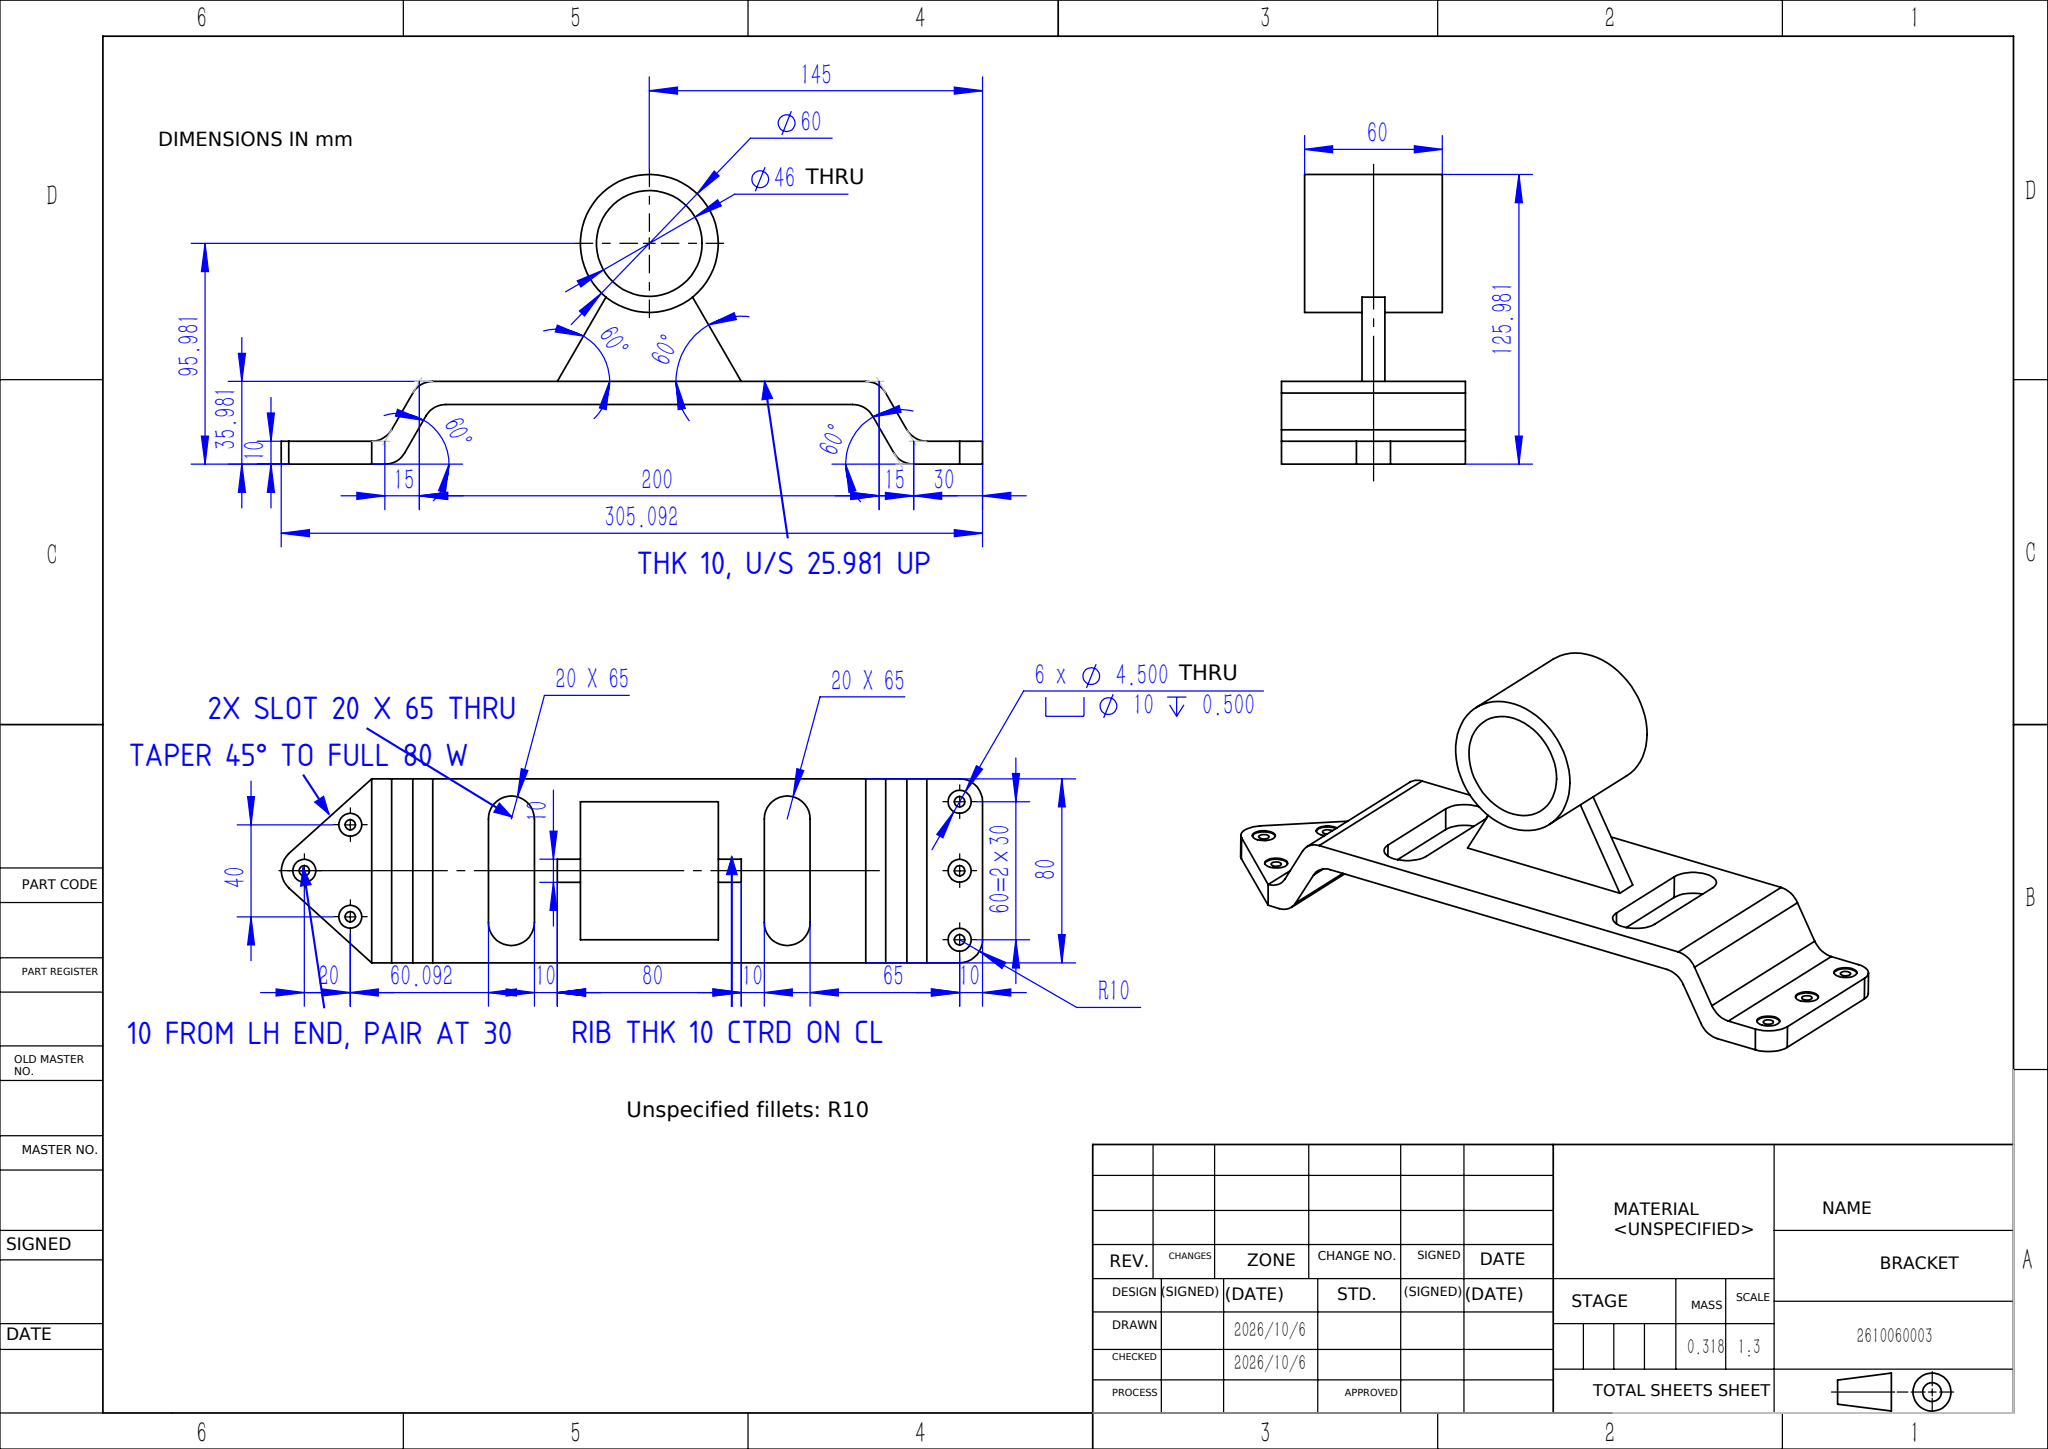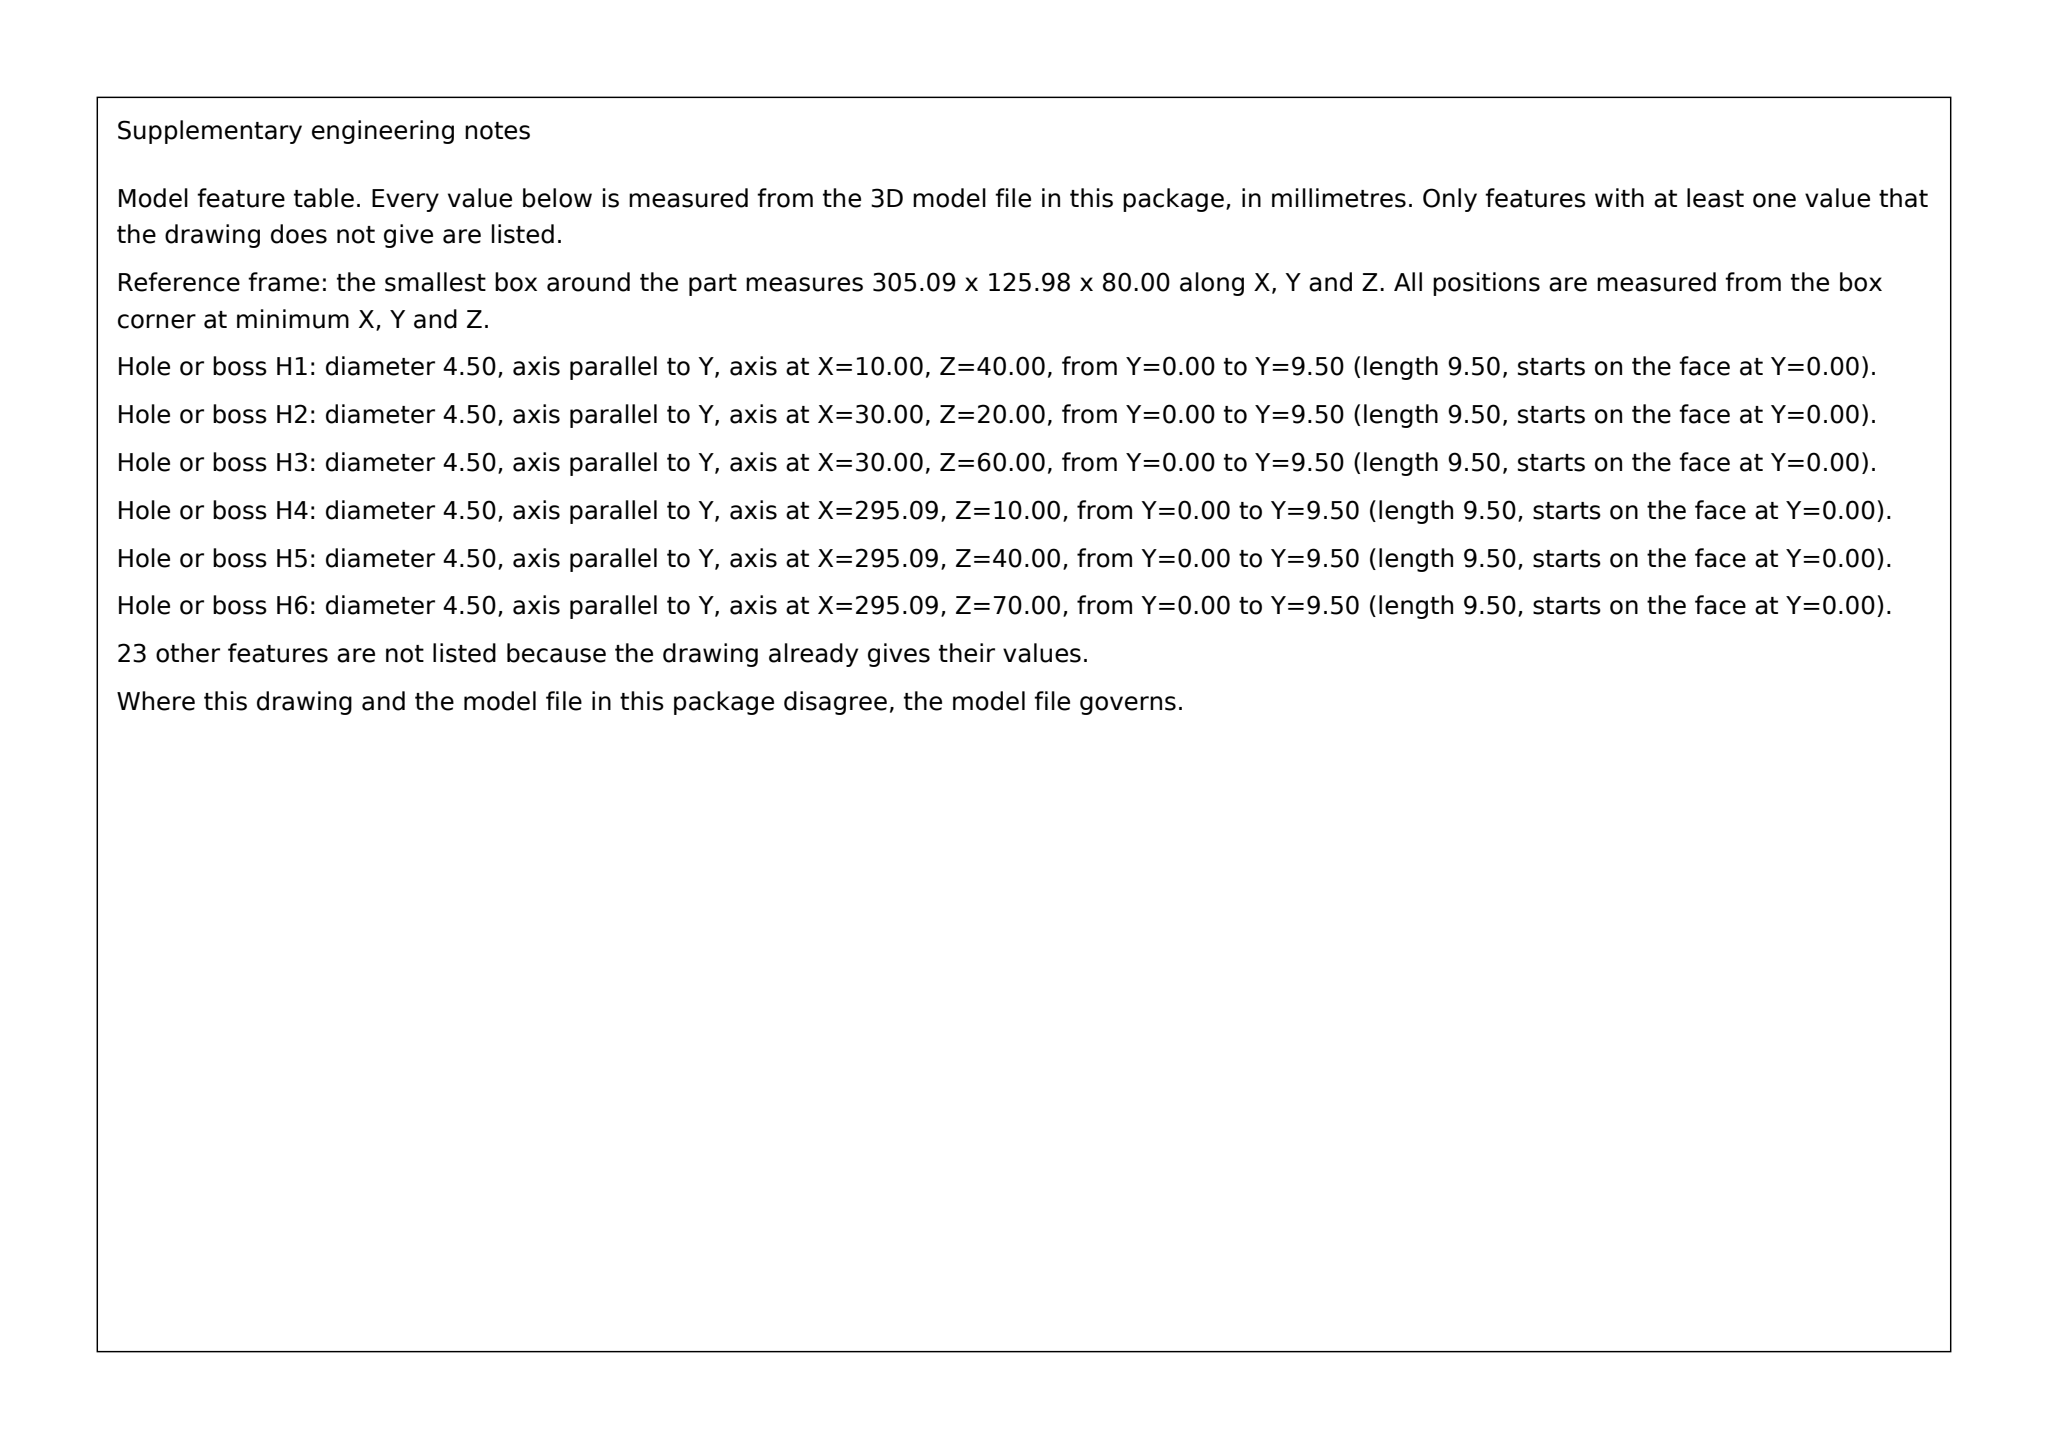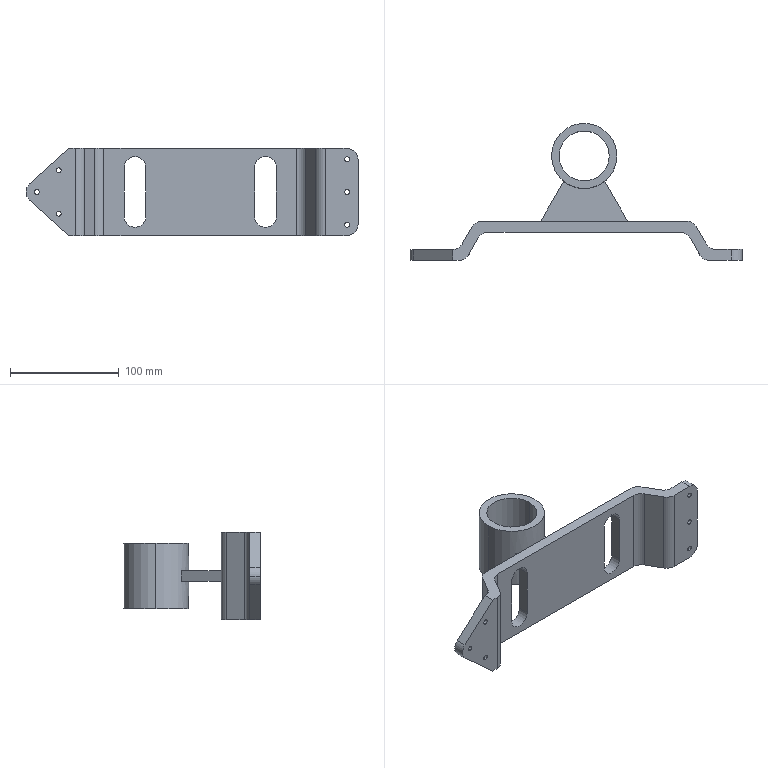Part | SolidWorks | mm | 1 solid | 77 faces | box 305.09 x 125.98 x 80 mm | volume 317970 mm3 | cylinder 46 | plane 31 | commonest cylinder face diameters 20 x18 10 x12 4.5 x12 46 x2 60 x2
Drawing notes:
BASE PLATE THK 10, UNDERSIDE 25.981 ABOVE PAD BOTTOM FACE | from the solid: y-planes at 25.98 and 35.98 (plate underside/top); end pads y 0-10
INCLINED SUPPORT RIB THK 10, CTRD ON 80 WIDTH CL | from the solid: z-planes at 35.0 and 45.0, symmetric about z=40 of 80 wide part
LEFT PAD TAPERS 45° EA SIDE OF CL TO FULL 80 W AT 35.86 FROM LH END | from the solid: Ø20 pads at x10,z40 and x30,z20/z60 (equal R10) give 45° tangent lines; edge reaches z=0/z=80 at x=35.86; body side planes z=0 & z=80
LH HOLE GRP: NOSE HOLE CL 10 FROM LH END, PAIR CL 30 FROM LH END | from the solid: Ø4.5 THRU cylinders at x=10.0 (z=40) and x=30.0 (z=20,60), measured from bbox x-min (left end, overall 305.092)
2X SLOT 20 X 65 THRU (10 THK FLANGE) | from the solid: Ø20 y-axis cyls at x=100.09 & 220.09, z=17.5/62.5, len 10; y planes 0 & 10 => thru 10 thk plate